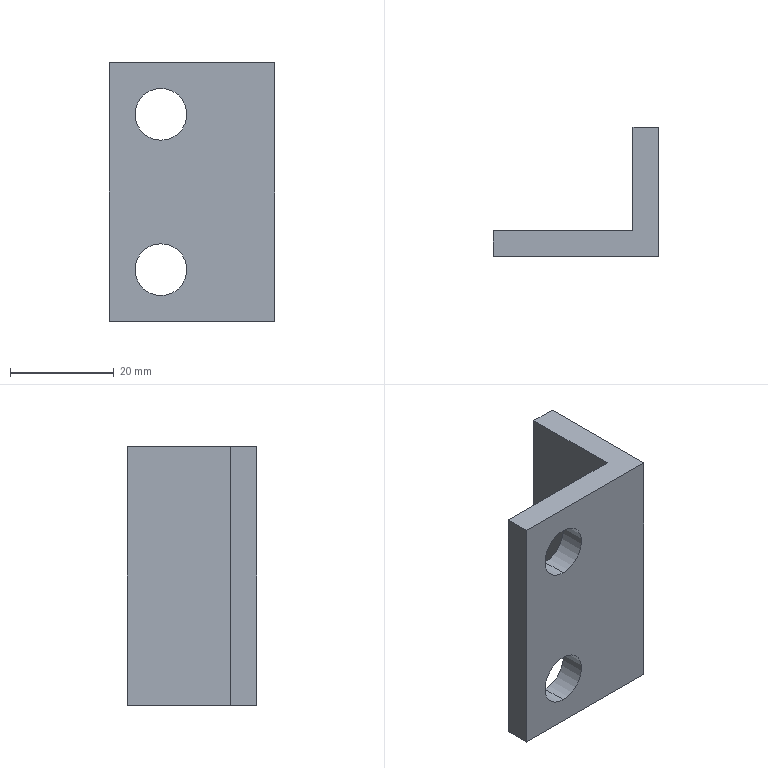Component | SolidWorks | 04-1 | 1 solid | 12 faces | box 32 x 25 x 50 mm | volume 12215 mm3 | plane 8 | cylinder 4 | commonest cylinder face diameters 10 x4
build123d program:
from build123d import *

# Parameters (mm, degrees)
BOSS_EXTRUDE1_DEPTH = 25
SKETCH2_R           = 5
CUT_EXTRUDE1_DEPTH  = 42.881


with BuildPart() as part:
    # Sketch1 → Boss-Extrude1 (new, symmetric)
    with BuildSketch(Plane.XY):
        Polygon((0, 0), (27, 0), (27, 5), (-5, 5), (-5, -20), (0, -20), align=None)
    extrude(amount=BOSS_EXTRUDE1_DEPTH, both=True)

    # Sketch2 → Cut-Extrude1 (cut, through all)
    with BuildSketch(Plane.XZ):
        with Locations(Location((17, 15, 0), (0, 0, 270))):
            Circle(SKETCH2_R)
        with Locations(Location((17, -15, 0), (0, 0, 270))):
            Circle(SKETCH2_R)
    extrude(amount=-CUT_EXTRUDE1_DEPTH, mode=Mode.SUBTRACT)


solid = part.part

# Placed as in the assembly
solid = solid.moved(Location((-25, 141.3, 101), (0, 0, 180)))
STEP:
#1=CARTESIAN_POINT('',(-1.654,5.366,3.583));
#2=VERTEX_POINT('',#1);
#3=CARTESIAN_POINT('',(-1.654,5.366,3.189));
#4=VERTEX_POINT('',#3);
#5=CARTESIAN_POINT('',(-1.654,5.366,3.386));
#6=DIRECTION('',(0.,1.,-0.));
#7=DIRECTION('',(0.,0.,-1.));
#8=AXIS2_PLACEMENT_3D('',#5,#6,#7);
#9=CIRCLE('',#8,0.1969);
#10=EDGE_CURVE('',#2,#4,#9,.T.);
#11=ORIENTED_EDGE('',*,*,#10,.F.);
#12=CARTESIAN_POINT('',(-1.654,5.563,3.583));
#13=VERTEX_POINT('',#12);
#14=CARTESIAN_POINT('',(-1.654,5.366,3.583));
#15=DIRECTION('',(0.,1.,-0.));
#16=VECTOR('',#15,39.37);
#17=LINE('',#14,#16);
#18=EDGE_CURVE('',#2,#13,#17,.T.);
#19=ORIENTED_EDGE('',*,*,#18,.T.);
#20=CARTESIAN_POINT('',(-1.654,5.563,3.189));
#21=VERTEX_POINT('',#20);
#22=CARTESIAN_POINT('',(-1.654,5.563,3.386));
#23=DIRECTION('',(0.,1.,-0.));
#24=DIRECTION('',(0.,0.,-1.));
#25=AXIS2_PLACEMENT_3D('',#22,#23,#24);
#26=CIRCLE('',#25,0.1969);
#27=EDGE_CURVE('',#13,#21,#26,.T.);
#28=ORIENTED_EDGE('',*,*,#27,.T.);
#29=CARTESIAN_POINT('',(-1.654,5.366,3.189));
#30=DIRECTION('',(0.,1.,-0.));
#31=VECTOR('',#30,39.37);
#32=LINE('',#29,#31);
#33=EDGE_CURVE('',#4,#21,#32,.T.);
#34=ORIENTED_EDGE('',*,*,#33,.F.);
#35=EDGE_LOOP('',(#11,#19,#28,#34));
#36=FACE_OUTER_BOUND('',#35,.T.);
#37=CARTESIAN_POINT('',(-1.654,5.366,3.386));
#38=DIRECTION('',(0.,1.,-0.));
#39=DIRECTION('',(0.,0.,-1.));
#40=AXIS2_PLACEMENT_3D('',#37,#38,#39);
#41=CYLINDRICAL_SURFACE('',#40,0.1969);
#42=ADVANCED_FACE('',(#36),#41,.F.);
#43=CARTESIAN_POINT('',(-1.654,5.366,4.764));
#44=VERTEX_POINT('',#43);
#45=CARTESIAN_POINT('',(-1.654,5.366,4.37));
#46=VERTEX_POINT('',#45);
#47=CARTESIAN_POINT('',(-1.654,5.366,4.567));
#48=DIRECTION('',(0.,1.,-0.));
#49=DIRECTION('',(0.,0.,-1.));
#50=AXIS2_PLACEMENT_3D('',#47,#48,#49);
#51=CIRCLE('',#50,0.1969);
#52=EDGE_CURVE('',#44,#46,#51,.T.);
#53=ORIENTED_EDGE('',*,*,#52,.F.);
#54=CARTESIAN_POINT('',(-1.654,5.563,4.764));
#55=VERTEX_POINT('',#54);
#56=CARTESIAN_POINT('',(-1.654,5.366,4.764));
#57=DIRECTION('',(0.,1.,-0.));
#58=VECTOR('',#57,39.37);
#59=LINE('',#56,#58);
#60=EDGE_CURVE('',#44,#55,#59,.T.);
#61=ORIENTED_EDGE('',*,*,#60,.T.);
#62=CARTESIAN_POINT('',(-1.654,5.563,4.37));
#63=VERTEX_POINT('',#62);
#64=CARTESIAN_POINT('',(-1.654,5.563,4.567));
#65=DIRECTION('',(0.,1.,-0.));
#66=DIRECTION('',(0.,0.,-1.));
#67=AXIS2_PLACEMENT_3D('',#64,#65,#66);
#68=CIRCLE('',#67,0.1969);
#69=EDGE_CURVE('',#55,#63,#68,.T.);
#70=ORIENTED_EDGE('',*,*,#69,.T.);
#71=CARTESIAN_POINT('',(-1.654,5.366,4.37));
#72=DIRECTION('',(0.,1.,-0.));
#73=VECTOR('',#72,39.37);
#74=LINE('',#71,#73);
#75=EDGE_CURVE('',#46,#63,#74,.T.);
#76=ORIENTED_EDGE('',*,*,#75,.F.);
#77=EDGE_LOOP('',(#53,#61,#70,#76));
#78=FACE_OUTER_BOUND('',#77,.T.);
#79=CARTESIAN_POINT('',(-1.654,5.366,4.567));
#80=DIRECTION('',(0.,1.,-0.));
#81=DIRECTION('',(0.,0.,-1.));
#82=AXIS2_PLACEMENT_3D('',#79,#80,#81);
#83=CYLINDRICAL_SURFACE('',#82,0.1969);
#84=ADVANCED_FACE('',(#78),#83,.F.);
#85=CARTESIAN_POINT('',(-0.9843,6.35,2.992));
#86=VERTEX_POINT('',#85);
#87=CARTESIAN_POINT('',(-0.9843,5.563,2.992));
#88=VERTEX_POINT('',#87);
#89=CARTESIAN_POINT('',(-0.9843,5.563,2.992));
#90=DIRECTION('',(0.,-1.,0.));
#91=VECTOR('',#90,39.37);
#92=LINE('',#89,#91);
#93=EDGE_CURVE('',#86,#88,#92,.T.);
#94=ORIENTED_EDGE('',*,*,#93,.T.);
#95=CARTESIAN_POINT('',(-0.9843,5.563,4.961));
#96=VERTEX_POINT('',#95);
#97=CARTESIAN_POINT('',(-0.9843,5.563,4.961));
#98=DIRECTION('',(0.,-0.,-1.));
#99=VECTOR('',#98,39.37);
#100=LINE('',#97,#99);
#101=EDGE_CURVE('',#96,#88,#100,.T.);
#102=ORIENTED_EDGE('',*,*,#101,.F.);
#103=CARTESIAN_POINT('',(-0.9843,6.35,4.961));
#104=VERTEX_POINT('',#103);
#105=CARTESIAN_POINT('',(-0.9843,5.563,4.961));
#106=DIRECTION('',(0.,-1.,0.));
#107=VECTOR('',#106,39.37);
#108=LINE('',#105,#107);
#109=EDGE_CURVE('',#104,#96,#108,.T.);
#110=ORIENTED_EDGE('',*,*,#109,.F.);
#111=CARTESIAN_POINT('',(-0.9843,6.35,4.961));
#112=DIRECTION('',(0.,-0.,-1.));
#113=VECTOR('',#112,39.37);
#114=LINE('',#111,#113);
#115=EDGE_CURVE('',#104,#86,#114,.T.);
#116=ORIENTED_EDGE('',*,*,#115,.T.);
#117=EDGE_LOOP('',(#94,#102,#110,#116));
#118=FACE_OUTER_BOUND('',#117,.T.);
#119=CARTESIAN_POINT('',(-0.9843,5.563,4.961));
#120=DIRECTION('',(1.,0.,0.));
#121=DIRECTION('',(-0.,1.,-0.));
#122=AXIS2_PLACEMENT_3D('',#119,#120,#121);
#123=PLANE('',#122);
#124=ADVANCED_FACE('',(#118),#123,.F.);
#125=CARTESIAN_POINT('',(-1.654,5.563,3.386));
#126=DIRECTION('',(0.,1.,-0.));
#127=DIRECTION('',(0.,0.,-1.));
#128=AXIS2_PLACEMENT_3D('',#125,#126,#127);
#129=CIRCLE('',#128,0.1969);
#130=EDGE_CURVE('',#21,#13,#129,.T.);
#131=ORIENTED_EDGE('',*,*,#130,.F.);
#132=ORIENTED_EDGE('',*,*,#27,.F.);
#133=EDGE_LOOP('',(#131,#132));
#134=FACE_BOUND('',#133,.T.);
#135=CARTESIAN_POINT('',(-1.654,5.563,4.567));
#136=DIRECTION('',(0.,1.,-0.));
#137=DIRECTION('',(0.,0.,-1.));
#138=AXIS2_PLACEMENT_3D('',#135,#136,#137);
#139=CIRCLE('',#138,0.1969);
#140=EDGE_CURVE('',#63,#55,#139,.T.);
#141=ORIENTED_EDGE('',*,*,#140,.F.);
#142=ORIENTED_EDGE('',*,*,#69,.F.);
#143=EDGE_LOOP('',(#141,#142));
#144=FACE_BOUND('',#143,.T.);
#145=CARTESIAN_POINT('',(-2.047,5.563,2.992));
#146=VERTEX_POINT('',#145);
#147=CARTESIAN_POINT('',(-0.9843,5.563,2.992));
#148=DIRECTION('',(-1.,0.,-0.));
#149=VECTOR('',#148,39.37);
#150=LINE('',#147,#149);
#151=EDGE_CURVE('',#88,#146,#150,.T.);
#152=ORIENTED_EDGE('',*,*,#151,.T.);
#153=CARTESIAN_POINT('',(-2.047,5.563,4.961));
#154=VERTEX_POINT('',#153);
#155=CARTESIAN_POINT('',(-2.047,5.563,4.961));
#156=DIRECTION('',(0.,-0.,-1.));
#157=VECTOR('',#156,39.37);
#158=LINE('',#155,#157);
#159=EDGE_CURVE('',#154,#146,#158,.T.);
#160=ORIENTED_EDGE('',*,*,#159,.F.);
#161=CARTESIAN_POINT('',(-0.9843,5.563,4.961));
#162=DIRECTION('',(-1.,0.,-0.));
#163=VECTOR('',#162,39.37);
#164=LINE('',#161,#163);
#165=EDGE_CURVE('',#96,#154,#164,.T.);
#166=ORIENTED_EDGE('',*,*,#165,.F.);
#167=ORIENTED_EDGE('',*,*,#101,.T.);
#168=EDGE_LOOP('',(#152,#160,#166,#167));
#169=FACE_OUTER_BOUND('',#168,.T.);
#170=CARTESIAN_POINT('',(-0.9843,5.563,4.961));
#171=DIRECTION('',(-0.,-1.,0.));
#172=DIRECTION('',(-0.,0.,1.));
#173=AXIS2_PLACEMENT_3D('',#170,#171,#172);
#174=PLANE('',#173);
#175=ADVANCED_FACE('',(#134,#144,#169),#174,.F.);
#176=CARTESIAN_POINT('',(-2.047,5.366,2.992));
#177=VERTEX_POINT('',#176);
#178=CARTESIAN_POINT('',(-2.047,5.563,2.992));
#179=DIRECTION('',(-0.,-1.,0.));
#180=VECTOR('',#179,39.37);
#181=LINE('',#178,#180);
#182=EDGE_CURVE('',#146,#177,#181,.T.);
#183=ORIENTED_EDGE('',*,*,#182,.T.);
#184=CARTESIAN_POINT('',(-2.047,5.366,4.961));
#185=VERTEX_POINT('',#184);
#186=CARTESIAN_POINT('',(-2.047,5.366,4.961));
#187=DIRECTION('',(0.,-0.,-1.));
#188=VECTOR('',#187,39.37);
#189=LINE('',#186,#188);
#190=EDGE_CURVE('',#185,#177,#189,.T.);
#191=ORIENTED_EDGE('',*,*,#190,.F.);
#192=CARTESIAN_POINT('',(-2.047,5.563,4.961));
#193=DIRECTION('',(-0.,-1.,0.));
#194=VECTOR('',#193,39.37);
#195=LINE('',#192,#194);
#196=EDGE_CURVE('',#154,#185,#195,.T.);
#197=ORIENTED_EDGE('',*,*,#196,.F.);
#198=ORIENTED_EDGE('',*,*,#159,.T.);
#199=EDGE_LOOP('',(#183,#191,#197,#198));
#200=FACE_OUTER_BOUND('',#199,.T.);
#201=CARTESIAN_POINT('',(-2.047,5.563,4.961));
#202=DIRECTION('',(1.,-0.,0.));
#203=DIRECTION('',(-0.,0.,1.));
#204=AXIS2_PLACEMENT_3D('',#201,#202,#203);
#205=PLANE('',#204);
#206=ADVANCED_FACE('',(#200),#205,.F.);
#207=CARTESIAN_POINT('',(-1.654,5.366,3.386));
#208=DIRECTION('',(0.,1.,-0.));
#209=DIRECTION('',(0.,0.,-1.));
#210=AXIS2_PLACEMENT_3D('',#207,#208,#209);
#211=CIRCLE('',#210,0.1969);
#212=EDGE_CURVE('',#4,#2,#211,.T.);
#213=ORIENTED_EDGE('',*,*,#212,.T.);
#214=ORIENTED_EDGE('',*,*,#10,.T.);
#215=EDGE_LOOP('',(#213,#214));
#216=FACE_BOUND('',#215,.T.);
#217=CARTESIAN_POINT('',(-1.654,5.366,4.567));
#218=DIRECTION('',(0.,1.,-0.));
#219=DIRECTION('',(0.,0.,-1.));
#220=AXIS2_PLACEMENT_3D('',#217,#218,#219);
#221=CIRCLE('',#220,0.1969);
#222=EDGE_CURVE('',#46,#44,#221,.T.);
#223=ORIENTED_EDGE('',*,*,#222,.T.);
#224=ORIENTED_EDGE('',*,*,#52,.T.);
#225=EDGE_LOOP('',(#223,#224));
#226=FACE_BOUND('',#225,.T.);
#227=CARTESIAN_POINT('',(-0.7874,5.366,2.992));
#228=VERTEX_POINT('',#227);
#229=CARTESIAN_POINT('',(-0.7874,5.366,2.992));
#230=DIRECTION('',(1.,-0.,0.));
#231=VECTOR('',#230,39.37);
#232=LINE('',#229,#231);
#233=EDGE_CURVE('',#177,#228,#232,.T.);
#234=ORIENTED_EDGE('',*,*,#233,.T.);
#235=CARTESIAN_POINT('',(-0.7874,5.366,4.961));
#236=VERTEX_POINT('',#235);
#237=CARTESIAN_POINT('',(-0.7874,5.366,4.961));
#238=DIRECTION('',(0.,-0.,-1.));
#239=VECTOR('',#238,39.37);
#240=LINE('',#237,#239);
#241=EDGE_CURVE('',#236,#228,#240,.T.);
#242=ORIENTED_EDGE('',*,*,#241,.F.);
#243=CARTESIAN_POINT('',(-0.7874,5.366,4.961));
#244=DIRECTION('',(1.,-0.,0.));
#245=VECTOR('',#244,39.37);
#246=LINE('',#243,#245);
#247=EDGE_CURVE('',#185,#236,#246,.T.);
#248=ORIENTED_EDGE('',*,*,#247,.F.);
#249=ORIENTED_EDGE('',*,*,#190,.T.);
#250=EDGE_LOOP('',(#234,#242,#248,#249));
#251=FACE_OUTER_BOUND('',#250,.T.);
#252=CARTESIAN_POINT('',(-0.7874,5.366,4.961));
#253=DIRECTION('',(0.,1.,-0.));
#254=DIRECTION('',(0.,-0.,-1.));
#255=AXIS2_PLACEMENT_3D('',#252,#253,#254);
#256=PLANE('',#255);
#257=ADVANCED_FACE('',(#216,#226,#251),#256,.F.);
#258=CARTESIAN_POINT('',(-0.7874,6.35,2.992));
#259=VERTEX_POINT('',#258);
#260=CARTESIAN_POINT('',(-0.7874,5.366,2.992));
#261=DIRECTION('',(-0.,1.,-0.));
#262=VECTOR('',#261,39.37);
#263=LINE('',#260,#262);
#264=EDGE_CURVE('',#228,#259,#263,.T.);
#265=ORIENTED_EDGE('',*,*,#264,.T.);
#266=CARTESIAN_POINT('',(-0.7874,6.35,4.961));
#267=VERTEX_POINT('',#266);
#268=CARTESIAN_POINT('',(-0.7874,6.35,4.961));
#269=DIRECTION('',(0.,-0.,-1.));
#270=VECTOR('',#269,39.37);
#271=LINE('',#268,#270);
#272=EDGE_CURVE('',#267,#259,#271,.T.);
#273=ORIENTED_EDGE('',*,*,#272,.F.);
#274=CARTESIAN_POINT('',(-0.7874,5.366,4.961));
#275=DIRECTION('',(-0.,1.,-0.));
#276=VECTOR('',#275,39.37);
#277=LINE('',#274,#276);
#278=EDGE_CURVE('',#236,#267,#277,.T.);
#279=ORIENTED_EDGE('',*,*,#278,.F.);
#280=ORIENTED_EDGE('',*,*,#241,.T.);
#281=EDGE_LOOP('',(#265,#273,#279,#280));
#282=FACE_OUTER_BOUND('',#281,.T.);
#283=CARTESIAN_POINT('',(-0.7874,5.366,4.961));
#284=DIRECTION('',(-1.,-0.,-0.));
#285=DIRECTION('',(0.,-1.,0.));
#286=AXIS2_PLACEMENT_3D('',#283,#284,#285);
#287=PLANE('',#286);
#288=ADVANCED_FACE('',(#282),#287,.F.);
#289=CARTESIAN_POINT('',(-0.7874,6.35,2.992));
#290=DIRECTION('',(-1.,0.,-0.));
#291=VECTOR('',#290,39.37);
#292=LINE('',#289,#291);
#293=EDGE_CURVE('',#259,#86,#292,.T.);
#294=ORIENTED_EDGE('',*,*,#293,.T.);
#295=ORIENTED_EDGE('',*,*,#115,.F.);
#296=CARTESIAN_POINT('',(-0.7874,6.35,4.961));
#297=DIRECTION('',(-1.,0.,-0.));
#298=VECTOR('',#297,39.37);
#299=LINE('',#296,#298);
#300=EDGE_CURVE('',#267,#104,#299,.T.);
#301=ORIENTED_EDGE('',*,*,#300,.F.);
#302=ORIENTED_EDGE('',*,*,#272,.T.);
#303=EDGE_LOOP('',(#294,#295,#301,#302));
#304=FACE_OUTER_BOUND('',#303,.T.);
#305=CARTESIAN_POINT('',(-0.7874,6.35,4.961));
#306=DIRECTION('',(-0.,-1.,0.));
#307=DIRECTION('',(-0.,0.,1.));
#308=AXIS2_PLACEMENT_3D('',#305,#306,#307);
#309=PLANE('',#308);
#310=ADVANCED_FACE('',(#304),#309,.F.);
#311=ORIENTED_EDGE('',*,*,#109,.T.);
#312=ORIENTED_EDGE('',*,*,#165,.T.);
#313=ORIENTED_EDGE('',*,*,#196,.T.);
#314=ORIENTED_EDGE('',*,*,#247,.T.);
#315=ORIENTED_EDGE('',*,*,#278,.T.);
#316=ORIENTED_EDGE('',*,*,#300,.T.);
#317=EDGE_LOOP('',(#311,#312,#313,#314,#315,#316));
#318=FACE_OUTER_BOUND('',#317,.T.);
#319=CARTESIAN_POINT('',(-0.9843,5.563,4.961));
#320=DIRECTION('',(-0.,0.,1.));
#321=DIRECTION('',(-1.,0.,-0.));
#322=AXIS2_PLACEMENT_3D('',#319,#320,#321);
#323=PLANE('',#322);
#324=ADVANCED_FACE('',(#318),#323,.T.);
#325=ORIENTED_EDGE('',*,*,#93,.F.);
#326=ORIENTED_EDGE('',*,*,#293,.F.);
#327=ORIENTED_EDGE('',*,*,#264,.F.);
#328=ORIENTED_EDGE('',*,*,#233,.F.);
#329=ORIENTED_EDGE('',*,*,#182,.F.);
#330=ORIENTED_EDGE('',*,*,#151,.F.);
#331=EDGE_LOOP('',(#325,#326,#327,#328,#329,#330));
#332=FACE_OUTER_BOUND('',#331,.T.);
#333=CARTESIAN_POINT('',(-0.9843,5.563,2.992));
#334=DIRECTION('',(-0.,0.,1.));
#335=DIRECTION('',(-1.,0.,-0.));
#336=AXIS2_PLACEMENT_3D('',#333,#334,#335);
#337=PLANE('',#336);
#338=ADVANCED_FACE('',(#332),#337,.F.);
#339=ORIENTED_EDGE('',*,*,#60,.F.);
#340=ORIENTED_EDGE('',*,*,#222,.F.);
#341=ORIENTED_EDGE('',*,*,#75,.T.);
#342=ORIENTED_EDGE('',*,*,#140,.T.);
#343=EDGE_LOOP('',(#339,#340,#341,#342));
#344=FACE_OUTER_BOUND('',#343,.T.);
#345=CARTESIAN_POINT('',(-1.654,5.366,4.567));
#346=DIRECTION('',(0.,1.,-0.));
#347=DIRECTION('',(0.,0.,-1.));
#348=AXIS2_PLACEMENT_3D('',#345,#346,#347);
#349=CYLINDRICAL_SURFACE('',#348,0.1969);
#350=ADVANCED_FACE('',(#344),#349,.F.);
#351=ORIENTED_EDGE('',*,*,#18,.F.);
#352=ORIENTED_EDGE('',*,*,#212,.F.);
#353=ORIENTED_EDGE('',*,*,#33,.T.);
#354=ORIENTED_EDGE('',*,*,#130,.T.);
#355=EDGE_LOOP('',(#351,#352,#353,#354));
#356=FACE_OUTER_BOUND('',#355,.T.);
#357=CARTESIAN_POINT('',(-1.654,5.366,3.386));
#358=DIRECTION('',(0.,1.,-0.));
#359=DIRECTION('',(0.,0.,-1.));
#360=AXIS2_PLACEMENT_3D('',#357,#358,#359);
#361=CYLINDRICAL_SURFACE('',#360,0.1969);
#362=ADVANCED_FACE('',(#356),#361,.F.);
#363=CLOSED_SHELL('',(#42,#84,#124,#175,#206,#257,#288,#310,#324,#338,#350,#362));
#364=MANIFOLD_SOLID_BREP('',#363);
#365=CARTESIAN_POINT('',(0.,0.,0.));
#366=DIRECTION('',(0.,0.,1.));
#367=DIRECTION('',(1.,0.,0.));
#368=AXIS2_PLACEMENT_3D('',#365,#366,#367);
#369=(LENGTH_UNIT()NAMED_UNIT(*)SI_UNIT($,.METRE.));
#370=LENGTH_MEASURE_WITH_UNIT(LENGTH_MEASURE(0.0254),#369);
#371=DIMENSIONAL_EXPONENTS(1.,0.,0.,0.,0.,0.,0.);
#372=(CONVERSION_BASED_UNIT('',#370)LENGTH_UNIT()NAMED_UNIT(#371));
#373=UNCERTAINTY_MEASURE_WITH_UNIT(LENGTH_MEASURE(0.00001),#372,'','');
#374=(NAMED_UNIT(*)PLANE_ANGLE_UNIT()SI_UNIT($,.RADIAN.));
#375=(NAMED_UNIT(*)SI_UNIT($,.STERADIAN.)SOLID_ANGLE_UNIT());
#376=(GEOMETRIC_REPRESENTATION_CONTEXT(3)GLOBAL_UNCERTAINTY_ASSIGNED_CONTEXT((#373))GLOBAL_UNIT_ASSIGNED_CONTEXT((#372,#374,#375))REPRESENTATION_CONTEXT('',''));
#377=ADVANCED_BREP_SHAPE_REPRESENTATION('',(#364,#368),#376);
#378=COLOUR_RGB('',0.7922,0.8196,0.9333);
#379=FILL_AREA_STYLE_COLOUR('',#378);
#380=FILL_AREA_STYLE('',(#379));
#381=SURFACE_STYLE_FILL_AREA(#380);
#382=SURFACE_SIDE_STYLE('',(#381));
#383=SURFACE_STYLE_USAGE(.BOTH.,#382);
#384=PRESENTATION_STYLE_ASSIGNMENT((#383));
#385=STYLED_ITEM('',(#384),#364);
#386=PRESENTATION_LAYER_ASSIGNMENT('','',(#385));
#387=(LENGTH_UNIT()NAMED_UNIT(*)SI_UNIT($,.METRE.));
#388=LENGTH_MEASURE_WITH_UNIT(LENGTH_MEASURE(0.0254),#387);
#389=DIMENSIONAL_EXPONENTS(1.,0.,0.,0.,0.,0.,0.);
#390=(CONVERSION_BASED_UNIT('',#388)LENGTH_UNIT()NAMED_UNIT(#389));
#391=UNCERTAINTY_MEASURE_WITH_UNIT(LENGTH_MEASURE(0.00001),#390,'','');
#392=(NAMED_UNIT(*)PLANE_ANGLE_UNIT()SI_UNIT($,.RADIAN.));
#393=(NAMED_UNIT(*)SI_UNIT($,.STERADIAN.)SOLID_ANGLE_UNIT());
#394=(GEOMETRIC_REPRESENTATION_CONTEXT(3)GLOBAL_UNCERTAINTY_ASSIGNED_CONTEXT((#391))GLOBAL_UNIT_ASSIGNED_CONTEXT((#390,#392,#393))REPRESENTATION_CONTEXT('',''));
#395=MECHANICAL_DESIGN_GEOMETRIC_PRESENTATION_REPRESENTATION('',(#385),#394);